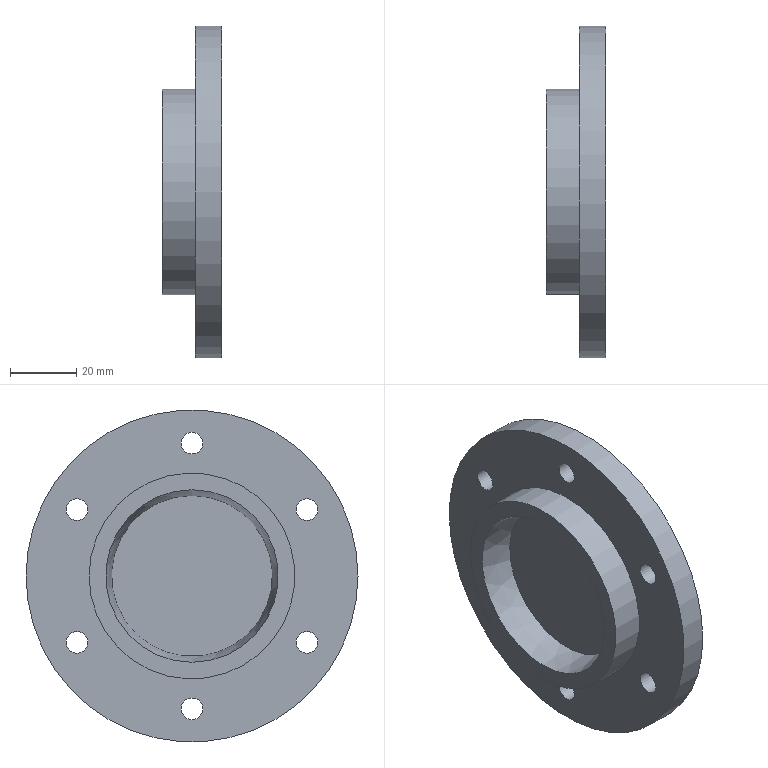Component | NX | DADUANMENGAI | 1 solid | 13 faces | box 18 x 100 x 100 mm | volume 71600 mm3 | cylinder 8 | plane 4 | cone 1 | commonest cylinder face diameters 6.5 x6 100 x1 62 x1
STEP:
#1=CARTESIAN_POINT('',(0.,0.,0.));
#2=DIRECTION('',(0.,0.,1.));
#3=DIRECTION('',(1.,0.,0.));
#4=AXIS2_PLACEMENT_3D('',#1,#2,#3);
#5=CARTESIAN_POINT('',(111.,234.641,-71.25));
#6=VERTEX_POINT('',#5);
#7=CARTESIAN_POINT('',(111.,234.641,-64.75));
#8=VERTEX_POINT('',#7);
#9=CARTESIAN_POINT('',(111.,234.641,-68.));
#10=DIRECTION('',(1.,0.,0.));
#11=DIRECTION('',(0.,0.,-1.));
#12=AXIS2_PLACEMENT_3D('',#9,#10,#11);
#13=CIRCLE('',#12,3.25);
#14=CARTESIAN_POINT('',(111.,200.,-88.));
#15=DIRECTION('',(1.,0.,0.));
#16=DIRECTION('',(0.,0.,-1.));
#17=AXIS2_PLACEMENT_3D('',#14,#15,#16);
#18=PLANE('',#17);
#19=CARTESIAN_POINT('',(-20.,34.641));
#20=DIRECTION('',(1.,0.));
#21=AXIS2_PLACEMENT_2D('',#19,#20);
#22=CIRCLE('',#21,3.25);
#23=(GEOMETRIC_REPRESENTATION_CONTEXT(2)PARAMETRIC_REPRESENTATION_CONTEXT()REPRESENTATION_CONTEXT('',''));
#24=DEFINITIONAL_REPRESENTATION('',(#22),#23);
#25=PCURVE('',#18,#24);
#26=CARTESIAN_POINT('',(119.,234.641,-68.));
#27=DIRECTION('',(-1.,0.,0.));
#28=DIRECTION('',(0.,0.,1.));
#29=AXIS2_PLACEMENT_3D('',#26,#27,#28);
#30=CYLINDRICAL_SURFACE('',#29,3.25);
#31=CARTESIAN_POINT('',(3.142,8.));
#32=DIRECTION('',(-1.,0.));
#33=VECTOR('',#32,1.);
#34=LINE('',#31,#33);
#35=(GEOMETRIC_REPRESENTATION_CONTEXT(2)PARAMETRIC_REPRESENTATION_CONTEXT()REPRESENTATION_CONTEXT('',''));
#36=DEFINITIONAL_REPRESENTATION('',(#34),#35);
#37=PCURVE('',#30,#36);
#38=SURFACE_CURVE('',#13,(#25,#37),.PCURVE_S1.);
#39=EDGE_CURVE('',#6,#8,#38,.T.);
#40=ORIENTED_EDGE('',*,*,#39,.T.);
#41=CARTESIAN_POINT('',(111.,234.641,-68.));
#42=DIRECTION('',(1.,0.,0.));
#43=DIRECTION('',(0.,0.,-1.));
#44=AXIS2_PLACEMENT_3D('',#41,#42,#43);
#45=CIRCLE('',#44,3.25);
#46=CARTESIAN_POINT('',(-20.,34.641));
#47=DIRECTION('',(1.,0.));
#48=AXIS2_PLACEMENT_2D('',#46,#47);
#49=CIRCLE('',#48,3.25);
#50=(GEOMETRIC_REPRESENTATION_CONTEXT(2)PARAMETRIC_REPRESENTATION_CONTEXT()REPRESENTATION_CONTEXT('',''));
#51=DEFINITIONAL_REPRESENTATION('',(#49),#50);
#52=PCURVE('',#18,#51);
#53=CARTESIAN_POINT('',(9.425,8.));
#54=DIRECTION('',(-1.,0.));
#55=VECTOR('',#54,1.);
#56=LINE('',#53,#55);
#57=(GEOMETRIC_REPRESENTATION_CONTEXT(2)PARAMETRIC_REPRESENTATION_CONTEXT()REPRESENTATION_CONTEXT('',''));
#58=DEFINITIONAL_REPRESENTATION('',(#56),#57);
#59=PCURVE('',#30,#58);
#60=SURFACE_CURVE('',#45,(#52,#59),.PCURVE_S1.);
#61=EDGE_CURVE('',#8,#6,#60,.T.);
#62=ORIENTED_EDGE('',*,*,#61,.T.);
#63=EDGE_LOOP('',(#40,#62));
#64=FACE_BOUND('',#63,.T.);
#65=CARTESIAN_POINT('',(111.,234.641,-111.25));
#66=VERTEX_POINT('',#65);
#67=CARTESIAN_POINT('',(111.,234.641,-104.75));
#68=VERTEX_POINT('',#67);
#69=CARTESIAN_POINT('',(111.,234.641,-108.));
#70=DIRECTION('',(1.,0.,0.));
#71=DIRECTION('',(0.,0.,-1.));
#72=AXIS2_PLACEMENT_3D('',#69,#70,#71);
#73=CIRCLE('',#72,3.25);
#74=CARTESIAN_POINT('',(20.,34.641));
#75=DIRECTION('',(1.,0.));
#76=AXIS2_PLACEMENT_2D('',#74,#75);
#77=CIRCLE('',#76,3.25);
#78=(GEOMETRIC_REPRESENTATION_CONTEXT(2)PARAMETRIC_REPRESENTATION_CONTEXT()REPRESENTATION_CONTEXT('',''));
#79=DEFINITIONAL_REPRESENTATION('',(#77),#78);
#80=PCURVE('',#18,#79);
#81=CARTESIAN_POINT('',(119.,234.641,-108.));
#82=DIRECTION('',(-1.,0.,0.));
#83=DIRECTION('',(0.,0.,1.));
#84=AXIS2_PLACEMENT_3D('',#81,#82,#83);
#85=CYLINDRICAL_SURFACE('',#84,3.25);
#86=CARTESIAN_POINT('',(3.142,8.));
#87=DIRECTION('',(-1.,0.));
#88=VECTOR('',#87,1.);
#89=LINE('',#86,#88);
#90=(GEOMETRIC_REPRESENTATION_CONTEXT(2)PARAMETRIC_REPRESENTATION_CONTEXT()REPRESENTATION_CONTEXT('',''));
#91=DEFINITIONAL_REPRESENTATION('',(#89),#90);
#92=PCURVE('',#85,#91);
#93=SURFACE_CURVE('',#73,(#80,#92),.PCURVE_S1.);
#94=EDGE_CURVE('',#66,#68,#93,.T.);
#95=ORIENTED_EDGE('',*,*,#94,.T.);
#96=CARTESIAN_POINT('',(111.,234.641,-108.));
#97=DIRECTION('',(1.,0.,0.));
#98=DIRECTION('',(0.,0.,-1.));
#99=AXIS2_PLACEMENT_3D('',#96,#97,#98);
#100=CIRCLE('',#99,3.25);
#101=CARTESIAN_POINT('',(20.,34.641));
#102=DIRECTION('',(1.,0.));
#103=AXIS2_PLACEMENT_2D('',#101,#102);
#104=CIRCLE('',#103,3.25);
#105=(GEOMETRIC_REPRESENTATION_CONTEXT(2)PARAMETRIC_REPRESENTATION_CONTEXT()REPRESENTATION_CONTEXT('',''));
#106=DEFINITIONAL_REPRESENTATION('',(#104),#105);
#107=PCURVE('',#18,#106);
#108=CARTESIAN_POINT('',(9.425,8.));
#109=DIRECTION('',(-1.,0.));
#110=VECTOR('',#109,1.);
#111=LINE('',#108,#110);
#112=(GEOMETRIC_REPRESENTATION_CONTEXT(2)PARAMETRIC_REPRESENTATION_CONTEXT()REPRESENTATION_CONTEXT('',''));
#113=DEFINITIONAL_REPRESENTATION('',(#111),#112);
#114=PCURVE('',#85,#113);
#115=SURFACE_CURVE('',#100,(#107,#114),.PCURVE_S1.);
#116=EDGE_CURVE('',#68,#66,#115,.T.);
#117=ORIENTED_EDGE('',*,*,#116,.T.);
#118=EDGE_LOOP('',(#95,#117));
#119=FACE_BOUND('',#118,.T.);
#120=CARTESIAN_POINT('',(111.,200.,-51.25));
#121=VERTEX_POINT('',#120);
#122=CARTESIAN_POINT('',(111.,200.,-44.75));
#123=VERTEX_POINT('',#122);
#124=CARTESIAN_POINT('',(111.,200.,-48.));
#125=DIRECTION('',(1.,0.,0.));
#126=DIRECTION('',(0.,0.,-1.));
#127=AXIS2_PLACEMENT_3D('',#124,#125,#126);
#128=CIRCLE('',#127,3.25);
#129=CARTESIAN_POINT('',(-40.,0.));
#130=DIRECTION('',(1.,0.));
#131=AXIS2_PLACEMENT_2D('',#129,#130);
#132=CIRCLE('',#131,3.25);
#133=(GEOMETRIC_REPRESENTATION_CONTEXT(2)PARAMETRIC_REPRESENTATION_CONTEXT()REPRESENTATION_CONTEXT('',''));
#134=DEFINITIONAL_REPRESENTATION('',(#132),#133);
#135=PCURVE('',#18,#134);
#136=CARTESIAN_POINT('',(119.,200.,-48.));
#137=DIRECTION('',(-1.,0.,0.));
#138=DIRECTION('',(0.,0.,1.));
#139=AXIS2_PLACEMENT_3D('',#136,#137,#138);
#140=CYLINDRICAL_SURFACE('',#139,3.25);
#141=CARTESIAN_POINT('',(3.142,8.));
#142=DIRECTION('',(-1.,0.));
#143=VECTOR('',#142,1.);
#144=LINE('',#141,#143);
#145=(GEOMETRIC_REPRESENTATION_CONTEXT(2)PARAMETRIC_REPRESENTATION_CONTEXT()REPRESENTATION_CONTEXT('',''));
#146=DEFINITIONAL_REPRESENTATION('',(#144),#145);
#147=PCURVE('',#140,#146);
#148=SURFACE_CURVE('',#128,(#135,#147),.PCURVE_S1.);
#149=EDGE_CURVE('',#121,#123,#148,.T.);
#150=ORIENTED_EDGE('',*,*,#149,.T.);
#151=CARTESIAN_POINT('',(111.,200.,-48.));
#152=DIRECTION('',(1.,0.,0.));
#153=DIRECTION('',(0.,0.,-1.));
#154=AXIS2_PLACEMENT_3D('',#151,#152,#153);
#155=CIRCLE('',#154,3.25);
#156=CARTESIAN_POINT('',(-40.,0.));
#157=DIRECTION('',(1.,0.));
#158=AXIS2_PLACEMENT_2D('',#156,#157);
#159=CIRCLE('',#158,3.25);
#160=(GEOMETRIC_REPRESENTATION_CONTEXT(2)PARAMETRIC_REPRESENTATION_CONTEXT()REPRESENTATION_CONTEXT('',''));
#161=DEFINITIONAL_REPRESENTATION('',(#159),#160);
#162=PCURVE('',#18,#161);
#163=CARTESIAN_POINT('',(9.425,8.));
#164=DIRECTION('',(-1.,0.));
#165=VECTOR('',#164,1.);
#166=LINE('',#163,#165);
#167=(GEOMETRIC_REPRESENTATION_CONTEXT(2)PARAMETRIC_REPRESENTATION_CONTEXT()REPRESENTATION_CONTEXT('',''));
#168=DEFINITIONAL_REPRESENTATION('',(#166),#167);
#169=PCURVE('',#140,#168);
#170=SURFACE_CURVE('',#155,(#162,#169),.PCURVE_S1.);
#171=EDGE_CURVE('',#123,#121,#170,.T.);
#172=ORIENTED_EDGE('',*,*,#171,.T.);
#173=EDGE_LOOP('',(#150,#172));
#174=FACE_BOUND('',#173,.T.);
#175=CARTESIAN_POINT('',(111.,200.,-131.25));
#176=VERTEX_POINT('',#175);
#177=CARTESIAN_POINT('',(111.,200.,-124.75));
#178=VERTEX_POINT('',#177);
#179=CARTESIAN_POINT('',(111.,200.,-128.));
#180=DIRECTION('',(1.,0.,0.));
#181=DIRECTION('',(0.,0.,-1.));
#182=AXIS2_PLACEMENT_3D('',#179,#180,#181);
#183=CIRCLE('',#182,3.25);
#184=CARTESIAN_POINT('',(40.,0.));
#185=DIRECTION('',(1.,0.));
#186=AXIS2_PLACEMENT_2D('',#184,#185);
#187=CIRCLE('',#186,3.25);
#188=(GEOMETRIC_REPRESENTATION_CONTEXT(2)PARAMETRIC_REPRESENTATION_CONTEXT()REPRESENTATION_CONTEXT('',''));
#189=DEFINITIONAL_REPRESENTATION('',(#187),#188);
#190=PCURVE('',#18,#189);
#191=CARTESIAN_POINT('',(119.,200.,-128.));
#192=DIRECTION('',(-1.,0.,0.));
#193=DIRECTION('',(0.,0.,1.));
#194=AXIS2_PLACEMENT_3D('',#191,#192,#193);
#195=CYLINDRICAL_SURFACE('',#194,3.25);
#196=CARTESIAN_POINT('',(3.142,8.));
#197=DIRECTION('',(-1.,0.));
#198=VECTOR('',#197,1.);
#199=LINE('',#196,#198);
#200=(GEOMETRIC_REPRESENTATION_CONTEXT(2)PARAMETRIC_REPRESENTATION_CONTEXT()REPRESENTATION_CONTEXT('',''));
#201=DEFINITIONAL_REPRESENTATION('',(#199),#200);
#202=PCURVE('',#195,#201);
#203=SURFACE_CURVE('',#183,(#190,#202),.PCURVE_S1.);
#204=EDGE_CURVE('',#176,#178,#203,.T.);
#205=ORIENTED_EDGE('',*,*,#204,.T.);
#206=CARTESIAN_POINT('',(111.,200.,-128.));
#207=DIRECTION('',(1.,0.,0.));
#208=DIRECTION('',(0.,0.,-1.));
#209=AXIS2_PLACEMENT_3D('',#206,#207,#208);
#210=CIRCLE('',#209,3.25);
#211=CARTESIAN_POINT('',(40.,0.));
#212=DIRECTION('',(1.,0.));
#213=AXIS2_PLACEMENT_2D('',#211,#212);
#214=CIRCLE('',#213,3.25);
#215=(GEOMETRIC_REPRESENTATION_CONTEXT(2)PARAMETRIC_REPRESENTATION_CONTEXT()REPRESENTATION_CONTEXT('',''));
#216=DEFINITIONAL_REPRESENTATION('',(#214),#215);
#217=PCURVE('',#18,#216);
#218=CARTESIAN_POINT('',(9.425,8.));
#219=DIRECTION('',(-1.,0.));
#220=VECTOR('',#219,1.);
#221=LINE('',#218,#220);
#222=(GEOMETRIC_REPRESENTATION_CONTEXT(2)PARAMETRIC_REPRESENTATION_CONTEXT()REPRESENTATION_CONTEXT('',''));
#223=DEFINITIONAL_REPRESENTATION('',(#221),#222);
#224=PCURVE('',#195,#223);
#225=SURFACE_CURVE('',#210,(#217,#224),.PCURVE_S1.);
#226=EDGE_CURVE('',#178,#176,#225,.T.);
#227=ORIENTED_EDGE('',*,*,#226,.T.);
#228=EDGE_LOOP('',(#205,#227));
#229=FACE_BOUND('',#228,.T.);
#230=CARTESIAN_POINT('',(111.,165.359,-71.25));
#231=VERTEX_POINT('',#230);
#232=CARTESIAN_POINT('',(111.,165.359,-64.75));
#233=VERTEX_POINT('',#232);
#234=CARTESIAN_POINT('',(111.,165.359,-68.));
#235=DIRECTION('',(1.,0.,0.));
#236=DIRECTION('',(0.,0.,-1.));
#237=AXIS2_PLACEMENT_3D('',#234,#235,#236);
#238=CIRCLE('',#237,3.25);
#239=CARTESIAN_POINT('',(-20.,-34.641));
#240=DIRECTION('',(1.,0.));
#241=AXIS2_PLACEMENT_2D('',#239,#240);
#242=CIRCLE('',#241,3.25);
#243=(GEOMETRIC_REPRESENTATION_CONTEXT(2)PARAMETRIC_REPRESENTATION_CONTEXT()REPRESENTATION_CONTEXT('',''));
#244=DEFINITIONAL_REPRESENTATION('',(#242),#243);
#245=PCURVE('',#18,#244);
#246=CARTESIAN_POINT('',(119.,165.359,-68.));
#247=DIRECTION('',(-1.,0.,0.));
#248=DIRECTION('',(0.,0.,1.));
#249=AXIS2_PLACEMENT_3D('',#246,#247,#248);
#250=CYLINDRICAL_SURFACE('',#249,3.25);
#251=CARTESIAN_POINT('',(3.142,8.));
#252=DIRECTION('',(-1.,0.));
#253=VECTOR('',#252,1.);
#254=LINE('',#251,#253);
#255=(GEOMETRIC_REPRESENTATION_CONTEXT(2)PARAMETRIC_REPRESENTATION_CONTEXT()REPRESENTATION_CONTEXT('',''));
#256=DEFINITIONAL_REPRESENTATION('',(#254),#255);
#257=PCURVE('',#250,#256);
#258=SURFACE_CURVE('',#238,(#245,#257),.PCURVE_S1.);
#259=EDGE_CURVE('',#231,#233,#258,.T.);
#260=ORIENTED_EDGE('',*,*,#259,.T.);
#261=CARTESIAN_POINT('',(111.,165.359,-68.));
#262=DIRECTION('',(1.,0.,0.));
#263=DIRECTION('',(0.,0.,-1.));
#264=AXIS2_PLACEMENT_3D('',#261,#262,#263);
#265=CIRCLE('',#264,3.25);
#266=CARTESIAN_POINT('',(-20.,-34.641));
#267=DIRECTION('',(1.,0.));
#268=AXIS2_PLACEMENT_2D('',#266,#267);
#269=CIRCLE('',#268,3.25);
#270=(GEOMETRIC_REPRESENTATION_CONTEXT(2)PARAMETRIC_REPRESENTATION_CONTEXT()REPRESENTATION_CONTEXT('',''));
#271=DEFINITIONAL_REPRESENTATION('',(#269),#270);
#272=PCURVE('',#18,#271);
#273=CARTESIAN_POINT('',(9.425,8.));
#274=DIRECTION('',(-1.,0.));
#275=VECTOR('',#274,1.);
#276=LINE('',#273,#275);
#277=(GEOMETRIC_REPRESENTATION_CONTEXT(2)PARAMETRIC_REPRESENTATION_CONTEXT()REPRESENTATION_CONTEXT('',''));
#278=DEFINITIONAL_REPRESENTATION('',(#276),#277);
#279=PCURVE('',#250,#278);
#280=SURFACE_CURVE('',#265,(#272,#279),.PCURVE_S1.);
#281=EDGE_CURVE('',#233,#231,#280,.T.);
#282=ORIENTED_EDGE('',*,*,#281,.T.);
#283=EDGE_LOOP('',(#260,#282));
#284=FACE_BOUND('',#283,.T.);
#285=CARTESIAN_POINT('',(111.,165.359,-111.25));
#286=VERTEX_POINT('',#285);
#287=CARTESIAN_POINT('',(111.,165.359,-104.75));
#288=VERTEX_POINT('',#287);
#289=CARTESIAN_POINT('',(111.,165.359,-108.));
#290=DIRECTION('',(1.,0.,0.));
#291=DIRECTION('',(0.,0.,-1.));
#292=AXIS2_PLACEMENT_3D('',#289,#290,#291);
#293=CIRCLE('',#292,3.25);
#294=CARTESIAN_POINT('',(20.,-34.641));
#295=DIRECTION('',(1.,0.));
#296=AXIS2_PLACEMENT_2D('',#294,#295);
#297=CIRCLE('',#296,3.25);
#298=(GEOMETRIC_REPRESENTATION_CONTEXT(2)PARAMETRIC_REPRESENTATION_CONTEXT()REPRESENTATION_CONTEXT('',''));
#299=DEFINITIONAL_REPRESENTATION('',(#297),#298);
#300=PCURVE('',#18,#299);
#301=CARTESIAN_POINT('',(119.,165.359,-108.));
#302=DIRECTION('',(-1.,0.,0.));
#303=DIRECTION('',(0.,0.,1.));
#304=AXIS2_PLACEMENT_3D('',#301,#302,#303);
#305=CYLINDRICAL_SURFACE('',#304,3.25);
#306=CARTESIAN_POINT('',(3.142,8.));
#307=DIRECTION('',(-1.,0.));
#308=VECTOR('',#307,1.);
#309=LINE('',#306,#308);
#310=(GEOMETRIC_REPRESENTATION_CONTEXT(2)PARAMETRIC_REPRESENTATION_CONTEXT()REPRESENTATION_CONTEXT('',''));
#311=DEFINITIONAL_REPRESENTATION('',(#309),#310);
#312=PCURVE('',#305,#311);
#313=SURFACE_CURVE('',#293,(#300,#312),.PCURVE_S1.);
#314=EDGE_CURVE('',#286,#288,#313,.T.);
#315=ORIENTED_EDGE('',*,*,#314,.T.);
#316=CARTESIAN_POINT('',(111.,165.359,-108.));
#317=DIRECTION('',(1.,0.,0.));
#318=DIRECTION('',(0.,0.,-1.));
#319=AXIS2_PLACEMENT_3D('',#316,#317,#318);
#320=CIRCLE('',#319,3.25);
#321=CARTESIAN_POINT('',(20.,-34.641));
#322=DIRECTION('',(1.,0.));
#323=AXIS2_PLACEMENT_2D('',#321,#322);
#324=CIRCLE('',#323,3.25);
#325=(GEOMETRIC_REPRESENTATION_CONTEXT(2)PARAMETRIC_REPRESENTATION_CONTEXT()REPRESENTATION_CONTEXT('',''));
#326=DEFINITIONAL_REPRESENTATION('',(#324),#325);
#327=PCURVE('',#18,#326);
#328=CARTESIAN_POINT('',(9.425,8.));
#329=DIRECTION('',(-1.,0.));
#330=VECTOR('',#329,1.);
#331=LINE('',#328,#330);
#332=(GEOMETRIC_REPRESENTATION_CONTEXT(2)PARAMETRIC_REPRESENTATION_CONTEXT()REPRESENTATION_CONTEXT('',''));
#333=DEFINITIONAL_REPRESENTATION('',(#331),#332);
#334=PCURVE('',#305,#333);
#335=SURFACE_CURVE('',#320,(#327,#334),.PCURVE_S1.);
#336=EDGE_CURVE('',#288,#286,#335,.T.);
#337=ORIENTED_EDGE('',*,*,#336,.T.);
#338=EDGE_LOOP('',(#315,#337));
#339=FACE_BOUND('',#338,.T.);
#340=CARTESIAN_POINT('',(111.,250.,-88.));
#341=VERTEX_POINT('',#340);
#342=CARTESIAN_POINT('',(111.,200.,-88.));
#343=DIRECTION('',(1.,0.,0.));
#344=DIRECTION('',(0.,1.,0.));
#345=AXIS2_PLACEMENT_3D('',#342,#343,#344);
#346=CIRCLE('',#345,50.);
#347=CARTESIAN_POINT('',(0.,0.));
#348=DIRECTION('',(0.,1.));
#349=AXIS2_PLACEMENT_2D('',#347,#348);
#350=CIRCLE('',#349,50.);
#351=(GEOMETRIC_REPRESENTATION_CONTEXT(2)PARAMETRIC_REPRESENTATION_CONTEXT()REPRESENTATION_CONTEXT('',''));
#352=DEFINITIONAL_REPRESENTATION('',(#350),#351);
#353=PCURVE('',#18,#352);
#354=CARTESIAN_POINT('',(119.,200.,-88.));
#355=DIRECTION('',(-1.,0.,0.));
#356=DIRECTION('',(0.,0.,1.));
#357=AXIS2_PLACEMENT_3D('',#354,#355,#356);
#358=CYLINDRICAL_SURFACE('',#357,50.);
#359=CARTESIAN_POINT('',(7.854,8.));
#360=DIRECTION('',(-1.,0.));
#361=VECTOR('',#360,1.);
#362=LINE('',#359,#361);
#363=(GEOMETRIC_REPRESENTATION_CONTEXT(2)PARAMETRIC_REPRESENTATION_CONTEXT()REPRESENTATION_CONTEXT('',''));
#364=DEFINITIONAL_REPRESENTATION('',(#362),#363);
#365=PCURVE('',#358,#364);
#366=SURFACE_CURVE('',#346,(#353,#365),.PCURVE_S1.);
#367=EDGE_CURVE('',#341,#341,#366,.T.);
#368=ORIENTED_EDGE('',*,*,#367,.F.);
#369=EDGE_LOOP('',(#368));
#370=FACE_BOUND('',#369,.T.);
#371=CARTESIAN_POINT('',(111.,231.,-88.));
#372=VERTEX_POINT('',#371);
#373=CARTESIAN_POINT('',(111.,200.,-88.));
#374=DIRECTION('',(-1.,0.,0.));
#375=DIRECTION('',(0.,1.,0.));
#376=AXIS2_PLACEMENT_3D('',#373,#374,#375);
#377=CIRCLE('',#376,31.);
#378=CARTESIAN_POINT('',(0.,31.));
#379=CARTESIAN_POINT('',(53.694,31.));
#380=CARTESIAN_POINT('',(26.847,-15.5));
#381=CARTESIAN_POINT('',(0.,-62.));
#382=CARTESIAN_POINT('',(-26.847,-15.5));
#383=CARTESIAN_POINT('',(-53.694,31.));
#384=CARTESIAN_POINT('',(0.,31.));
#385=(BOUNDED_CURVE()B_SPLINE_CURVE(2,(#378,#379,#380,#381,#382,#383,#384),.UNSPECIFIED.,.T.,.F.)B_SPLINE_CURVE_WITH_KNOTS((1,2,2,2,2,1),(-2.094,0.,2.094,4.189,6.283,8.378),.UNSPECIFIED.)CURVE()GEOMETRIC_REPRESENTATION_ITEM()RATIONAL_B_SPLINE_CURVE((1.,0.5,1.,0.5,1.,0.5,1.))REPRESENTATION_ITEM(''));
#386=(GEOMETRIC_REPRESENTATION_CONTEXT(2)PARAMETRIC_REPRESENTATION_CONTEXT()REPRESENTATION_CONTEXT('',''));
#387=DEFINITIONAL_REPRESENTATION('',(#385),#386);
#388=PCURVE('',#18,#387);
#389=CARTESIAN_POINT('',(101.,200.,-88.));
#390=DIRECTION('',(1.,0.,0.));
#391=DIRECTION('',(0.,0.,-1.));
#392=AXIS2_PLACEMENT_3D('',#389,#390,#391);
#393=CYLINDRICAL_SURFACE('',#392,31.);
#394=CARTESIAN_POINT('',(7.854,10.));
#395=DIRECTION('',(-1.,0.));
#396=VECTOR('',#395,1.);
#397=LINE('',#394,#396);
#398=(GEOMETRIC_REPRESENTATION_CONTEXT(2)PARAMETRIC_REPRESENTATION_CONTEXT()REPRESENTATION_CONTEXT('',''));
#399=DEFINITIONAL_REPRESENTATION('',(#397),#398);
#400=PCURVE('',#393,#399);
#401=SURFACE_CURVE('',#377,(#388,#400),.PCURVE_S1.);
#402=EDGE_CURVE('',#372,#372,#401,.T.);
#403=ORIENTED_EDGE('',*,*,#402,.F.);
#404=EDGE_LOOP('',(#403));
#405=FACE_BOUND('',#404,.T.);
#406=ADVANCED_FACE('',(#64,#119,#174,#229,#284,#339,#370,#405),#18,.F.);
#407=CARTESIAN_POINT('',(119.,250.,-88.));
#408=VERTEX_POINT('',#407);
#409=CARTESIAN_POINT('',(119.,200.,-88.));
#410=DIRECTION('',(1.,0.,0.));
#411=DIRECTION('',(0.,1.,0.));
#412=AXIS2_PLACEMENT_3D('',#409,#410,#411);
#413=CIRCLE('',#412,50.);
#414=CARTESIAN_POINT('',(7.854,0.));
#415=DIRECTION('',(-1.,0.));
#416=VECTOR('',#415,1.);
#417=LINE('',#414,#416);
#418=(GEOMETRIC_REPRESENTATION_CONTEXT(2)PARAMETRIC_REPRESENTATION_CONTEXT()REPRESENTATION_CONTEXT('',''));
#419=DEFINITIONAL_REPRESENTATION('',(#417),#418);
#420=PCURVE('',#358,#419);
#421=CARTESIAN_POINT('',(119.,200.,-88.));
#422=DIRECTION('',(1.,0.,0.));
#423=DIRECTION('',(0.,0.,-1.));
#424=AXIS2_PLACEMENT_3D('',#421,#422,#423);
#425=PLANE('',#424);
#426=CARTESIAN_POINT('',(0.,0.));
#427=DIRECTION('',(0.,1.));
#428=AXIS2_PLACEMENT_2D('',#426,#427);
#429=CIRCLE('',#428,50.);
#430=(GEOMETRIC_REPRESENTATION_CONTEXT(2)PARAMETRIC_REPRESENTATION_CONTEXT()REPRESENTATION_CONTEXT('',''));
#431=DEFINITIONAL_REPRESENTATION('',(#429),#430);
#432=PCURVE('',#425,#431);
#433=SURFACE_CURVE('',#413,(#420,#432),.PCURVE_S1.);
#434=EDGE_CURVE('',#408,#408,#433,.T.);
#435=ORIENTED_EDGE('',*,*,#434,.F.);
#436=CARTESIAN_POINT('',(119.,250.,-88.));
#437=CARTESIAN_POINT('',(111.,250.,-88.));
#438=B_SPLINE_CURVE_WITH_KNOTS('',1,(#436,#437),.UNSPECIFIED.,.F.,.F.,(2,2),(0.,8.),.PIECEWISE_BEZIER_KNOTS.);
#439=CARTESIAN_POINT('',(7.854,0.));
#440=DIRECTION('',(0.,1.));
#441=VECTOR('',#440,1.);
#442=LINE('',#439,#441);
#443=(GEOMETRIC_REPRESENTATION_CONTEXT(2)PARAMETRIC_REPRESENTATION_CONTEXT()REPRESENTATION_CONTEXT('',''));
#444=DEFINITIONAL_REPRESENTATION('',(#442),#443);
#445=PCURVE('',#358,#444);
#446=CARTESIAN_POINT('',(1.571,0.));
#447=DIRECTION('',(0.,1.));
#448=VECTOR('',#447,1.);
#449=LINE('',#446,#448);
#450=(GEOMETRIC_REPRESENTATION_CONTEXT(2)PARAMETRIC_REPRESENTATION_CONTEXT()REPRESENTATION_CONTEXT('',''));
#451=DEFINITIONAL_REPRESENTATION('',(#449),#450);
#452=PCURVE('',#358,#451);
#453=SEAM_CURVE('',#438,(#445,#452),.PCURVE_S1.);
#454=EDGE_CURVE('',#408,#341,#453,.T.);
#455=ORIENTED_EDGE('',*,*,#454,.T.);
#456=ORIENTED_EDGE('',*,*,#367,.T.);
#457=ORIENTED_EDGE('',*,*,#454,.F.);
#458=EDGE_LOOP('',(#435,#455,#456,#457));
#459=FACE_BOUND('',#458,.T.);
#460=ADVANCED_FACE('',(#459),#358,.T.);
#461=CARTESIAN_POINT('',(119.,234.641,-64.75));
#462=VERTEX_POINT('',#461);
#463=CARTESIAN_POINT('',(119.,234.641,-68.));
#464=DIRECTION('',(-1.,0.,0.));
#465=DIRECTION('',(0.,0.,1.));
#466=AXIS2_PLACEMENT_3D('',#463,#464,#465);
#467=CIRCLE('',#466,3.25);
#468=CARTESIAN_POINT('',(-23.25,34.641));
#469=CARTESIAN_POINT('',(-23.25,40.27));
#470=CARTESIAN_POINT('',(-18.375,37.456));
#471=CARTESIAN_POINT('',(-13.5,34.641));
#472=CARTESIAN_POINT('',(-18.375,31.826));
#473=CARTESIAN_POINT('',(-23.25,29.012));
#474=CARTESIAN_POINT('',(-23.25,34.641));
#475=(BOUNDED_CURVE()B_SPLINE_CURVE(2,(#468,#469,#470,#471,#472,#473,#474),.UNSPECIFIED.,.T.,.F.)B_SPLINE_CURVE_WITH_KNOTS((1,2,2,2,2,1),(-2.094,0.,2.094,4.189,6.283,8.378),.UNSPECIFIED.)CURVE()GEOMETRIC_REPRESENTATION_ITEM()RATIONAL_B_SPLINE_CURVE((1.,0.5,1.,0.5,1.,0.5,1.))REPRESENTATION_ITEM(''));
#476=(GEOMETRIC_REPRESENTATION_CONTEXT(2)PARAMETRIC_REPRESENTATION_CONTEXT()REPRESENTATION_CONTEXT('',''));
#477=DEFINITIONAL_REPRESENTATION('',(#475),#476);
#478=PCURVE('',#425,#477);
#479=CARTESIAN_POINT('',(0.,0.));
#480=DIRECTION('',(1.,0.));
#481=VECTOR('',#480,1.);
#482=LINE('',#479,#481);
#483=(GEOMETRIC_REPRESENTATION_CONTEXT(2)PARAMETRIC_REPRESENTATION_CONTEXT()REPRESENTATION_CONTEXT('',''));
#484=DEFINITIONAL_REPRESENTATION('',(#482),#483);
#485=PCURVE('',#30,#484);
#486=SURFACE_CURVE('',#467,(#478,#485),.PCURVE_S1.);
#487=EDGE_CURVE('',#462,#462,#486,.T.);
#488=ORIENTED_EDGE('',*,*,#487,.T.);
#489=EDGE_LOOP('',(#488));
#490=FACE_BOUND('',#489,.T.);
#491=CARTESIAN_POINT('',(119.,234.641,-104.75));
#492=VERTEX_POINT('',#491);
#493=CARTESIAN_POINT('',(119.,234.641,-108.));
#494=DIRECTION('',(-1.,0.,0.));
#495=DIRECTION('',(0.,0.,1.));
#496=AXIS2_PLACEMENT_3D('',#493,#494,#495);
#497=CIRCLE('',#496,3.25);
#498=CARTESIAN_POINT('',(16.75,34.641));
#499=CARTESIAN_POINT('',(16.75,40.27));
#500=CARTESIAN_POINT('',(21.625,37.456));
#501=CARTESIAN_POINT('',(26.5,34.641));
#502=CARTESIAN_POINT('',(21.625,31.826));
#503=CARTESIAN_POINT('',(16.75,29.012));
#504=CARTESIAN_POINT('',(16.75,34.641));
#505=(BOUNDED_CURVE()B_SPLINE_CURVE(2,(#498,#499,#500,#501,#502,#503,#504),.UNSPECIFIED.,.T.,.F.)B_SPLINE_CURVE_WITH_KNOTS((1,2,2,2,2,1),(-2.094,0.,2.094,4.189,6.283,8.378),.UNSPECIFIED.)CURVE()GEOMETRIC_REPRESENTATION_ITEM()RATIONAL_B_SPLINE_CURVE((1.,0.5,1.,0.5,1.,0.5,1.))REPRESENTATION_ITEM(''));
#506=(GEOMETRIC_REPRESENTATION_CONTEXT(2)PARAMETRIC_REPRESENTATION_CONTEXT()REPRESENTATION_CONTEXT('',''));
#507=DEFINITIONAL_REPRESENTATION('',(#505),#506);
#508=PCURVE('',#425,#507);
#509=CARTESIAN_POINT('',(0.,0.));
#510=DIRECTION('',(1.,0.));
#511=VECTOR('',#510,1.);
#512=LINE('',#509,#511);
#513=(GEOMETRIC_REPRESENTATION_CONTEXT(2)PARAMETRIC_REPRESENTATION_CONTEXT()REPRESENTATION_CONTEXT('',''));
#514=DEFINITIONAL_REPRESENTATION('',(#512),#513);
#515=PCURVE('',#85,#514);
#516=SURFACE_CURVE('',#497,(#508,#515),.PCURVE_S1.);
#517=EDGE_CURVE('',#492,#492,#516,.T.);
#518=ORIENTED_EDGE('',*,*,#517,.T.);
#519=EDGE_LOOP('',(#518));
#520=FACE_BOUND('',#519,.T.);
#521=CARTESIAN_POINT('',(119.,200.,-44.75));
#522=VERTEX_POINT('',#521);
#523=CARTESIAN_POINT('',(119.,200.,-48.));
#524=DIRECTION('',(-1.,0.,0.));
#525=DIRECTION('',(0.,0.,1.));
#526=AXIS2_PLACEMENT_3D('',#523,#524,#525);
#527=CIRCLE('',#526,3.25);
#528=CARTESIAN_POINT('',(-43.25,0.));
#529=CARTESIAN_POINT('',(-43.25,5.629));
#530=CARTESIAN_POINT('',(-38.375,2.815));
#531=CARTESIAN_POINT('',(-33.5,0.));
#532=CARTESIAN_POINT('',(-38.375,-2.815));
#533=CARTESIAN_POINT('',(-43.25,-5.629));
#534=CARTESIAN_POINT('',(-43.25,0.));
#535=(BOUNDED_CURVE()B_SPLINE_CURVE(2,(#528,#529,#530,#531,#532,#533,#534),.UNSPECIFIED.,.T.,.F.)B_SPLINE_CURVE_WITH_KNOTS((1,2,2,2,2,1),(-2.094,0.,2.094,4.189,6.283,8.378),.UNSPECIFIED.)CURVE()GEOMETRIC_REPRESENTATION_ITEM()RATIONAL_B_SPLINE_CURVE((1.,0.5,1.,0.5,1.,0.5,1.))REPRESENTATION_ITEM(''));
#536=(GEOMETRIC_REPRESENTATION_CONTEXT(2)PARAMETRIC_REPRESENTATION_CONTEXT()REPRESENTATION_CONTEXT('',''));
#537=DEFINITIONAL_REPRESENTATION('',(#535),#536);
#538=PCURVE('',#425,#537);
#539=CARTESIAN_POINT('',(0.,0.));
#540=DIRECTION('',(1.,0.));
#541=VECTOR('',#540,1.);
#542=LINE('',#539,#541);
#543=(GEOMETRIC_REPRESENTATION_CONTEXT(2)PARAMETRIC_REPRESENTATION_CONTEXT()REPRESENTATION_CONTEXT('',''));
#544=DEFINITIONAL_REPRESENTATION('',(#542),#543);
#545=PCURVE('',#140,#544);
#546=SURFACE_CURVE('',#527,(#538,#545),.PCURVE_S1.);
#547=EDGE_CURVE('',#522,#522,#546,.T.);
#548=ORIENTED_EDGE('',*,*,#547,.T.);
#549=EDGE_LOOP('',(#548));
#550=FACE_BOUND('',#549,.T.);
#551=CARTESIAN_POINT('',(119.,200.,-124.75));
#552=VERTEX_POINT('',#551);
#553=CARTESIAN_POINT('',(119.,200.,-128.));
#554=DIRECTION('',(-1.,0.,0.));
#555=DIRECTION('',(0.,0.,1.));
#556=AXIS2_PLACEMENT_3D('',#553,#554,#555);
#557=CIRCLE('',#556,3.25);
#558=CARTESIAN_POINT('',(36.75,0.));
#559=CARTESIAN_POINT('',(36.75,5.629));
#560=CARTESIAN_POINT('',(41.625,2.815));
#561=CARTESIAN_POINT('',(46.5,0.));
#562=CARTESIAN_POINT('',(41.625,-2.815));
#563=CARTESIAN_POINT('',(36.75,-5.629));
#564=CARTESIAN_POINT('',(36.75,0.));
#565=(BOUNDED_CURVE()B_SPLINE_CURVE(2,(#558,#559,#560,#561,#562,#563,#564),.UNSPECIFIED.,.T.,.F.)B_SPLINE_CURVE_WITH_KNOTS((1,2,2,2,2,1),(-2.094,0.,2.094,4.189,6.283,8.378),.UNSPECIFIED.)CURVE()GEOMETRIC_REPRESENTATION_ITEM()RATIONAL_B_SPLINE_CURVE((1.,0.5,1.,0.5,1.,0.5,1.))REPRESENTATION_ITEM(''));
#566=(GEOMETRIC_REPRESENTATION_CONTEXT(2)PARAMETRIC_REPRESENTATION_CONTEXT()REPRESENTATION_CONTEXT('',''));
#567=DEFINITIONAL_REPRESENTATION('',(#565),#566);
#568=PCURVE('',#425,#567);
#569=CARTESIAN_POINT('',(0.,0.));
#570=DIRECTION('',(1.,0.));
#571=VECTOR('',#570,1.);
#572=LINE('',#569,#571);
#573=(GEOMETRIC_REPRESENTATION_CONTEXT(2)PARAMETRIC_REPRESENTATION_CONTEXT()REPRESENTATION_CONTEXT('',''));
#574=DEFINITIONAL_REPRESENTATION('',(#572),#573);
#575=PCURVE('',#195,#574);
#576=SURFACE_CURVE('',#557,(#568,#575),.PCURVE_S1.);
#577=EDGE_CURVE('',#552,#552,#576,.T.);
#578=ORIENTED_EDGE('',*,*,#577,.T.);
#579=EDGE_LOOP('',(#578));
#580=FACE_BOUND('',#579,.T.);
#581=CARTESIAN_POINT('',(119.,165.359,-64.75));
#582=VERTEX_POINT('',#581);
#583=CARTESIAN_POINT('',(119.,165.359,-68.));
#584=DIRECTION('',(-1.,0.,0.));
#585=DIRECTION('',(0.,0.,1.));
#586=AXIS2_PLACEMENT_3D('',#583,#584,#585);
#587=CIRCLE('',#586,3.25);
#588=CARTESIAN_POINT('',(-23.25,-34.641));
#589=CARTESIAN_POINT('',(-23.25,-29.012));
#590=CARTESIAN_POINT('',(-18.375,-31.826));
#591=CARTESIAN_POINT('',(-13.5,-34.641));
#592=CARTESIAN_POINT('',(-18.375,-37.456));
#593=CARTESIAN_POINT('',(-23.25,-40.27));
#594=CARTESIAN_POINT('',(-23.25,-34.641));
#595=(BOUNDED_CURVE()B_SPLINE_CURVE(2,(#588,#589,#590,#591,#592,#593,#594),.UNSPECIFIED.,.T.,.F.)B_SPLINE_CURVE_WITH_KNOTS((1,2,2,2,2,1),(-2.094,0.,2.094,4.189,6.283,8.378),.UNSPECIFIED.)CURVE()GEOMETRIC_REPRESENTATION_ITEM()RATIONAL_B_SPLINE_CURVE((1.,0.5,1.,0.5,1.,0.5,1.))REPRESENTATION_ITEM(''));
#596=(GEOMETRIC_REPRESENTATION_CONTEXT(2)PARAMETRIC_REPRESENTATION_CONTEXT()REPRESENTATION_CONTEXT('',''));
#597=DEFINITIONAL_REPRESENTATION('',(#595),#596);
#598=PCURVE('',#425,#597);
#599=CARTESIAN_POINT('',(0.,0.));
#600=DIRECTION('',(1.,0.));
#601=VECTOR('',#600,1.);
#602=LINE('',#599,#601);
#603=(GEOMETRIC_REPRESENTATION_CONTEXT(2)PARAMETRIC_REPRESENTATION_CONTEXT()REPRESENTATION_CONTEXT('',''));
#604=DEFINITIONAL_REPRESENTATION('',(#602),#603);
#605=PCURVE('',#250,#604);
#606=SURFACE_CURVE('',#587,(#598,#605),.PCURVE_S1.);
#607=EDGE_CURVE('',#582,#582,#606,.T.);
#608=ORIENTED_EDGE('',*,*,#607,.T.);
#609=EDGE_LOOP('',(#608));
#610=FACE_BOUND('',#609,.T.);
#611=CARTESIAN_POINT('',(119.,165.359,-104.75));
#612=VERTEX_POINT('',#611);
#613=CARTESIAN_POINT('',(119.,165.359,-108.));
#614=DIRECTION('',(-1.,0.,0.));
#615=DIRECTION('',(0.,0.,1.));
#616=AXIS2_PLACEMENT_3D('',#613,#614,#615);
#617=CIRCLE('',#616,3.25);
#618=CARTESIAN_POINT('',(16.75,-34.641));
#619=CARTESIAN_POINT('',(16.75,-29.012));
#620=CARTESIAN_POINT('',(21.625,-31.826));
#621=CARTESIAN_POINT('',(26.5,-34.641));
#622=CARTESIAN_POINT('',(21.625,-37.456));
#623=CARTESIAN_POINT('',(16.75,-40.27));
#624=CARTESIAN_POINT('',(16.75,-34.641));
#625=(BOUNDED_CURVE()B_SPLINE_CURVE(2,(#618,#619,#620,#621,#622,#623,#624),.UNSPECIFIED.,.T.,.F.)B_SPLINE_CURVE_WITH_KNOTS((1,2,2,2,2,1),(-2.094,0.,2.094,4.189,6.283,8.378),.UNSPECIFIED.)CURVE()GEOMETRIC_REPRESENTATION_ITEM()RATIONAL_B_SPLINE_CURVE((1.,0.5,1.,0.5,1.,0.5,1.))REPRESENTATION_ITEM(''));
#626=(GEOMETRIC_REPRESENTATION_CONTEXT(2)PARAMETRIC_REPRESENTATION_CONTEXT()REPRESENTATION_CONTEXT('',''));
#627=DEFINITIONAL_REPRESENTATION('',(#625),#626);
#628=PCURVE('',#425,#627);
#629=CARTESIAN_POINT('',(0.,0.));
#630=DIRECTION('',(1.,0.));
#631=VECTOR('',#630,1.);
#632=LINE('',#629,#631);
#633=(GEOMETRIC_REPRESENTATION_CONTEXT(2)PARAMETRIC_REPRESENTATION_CONTEXT()REPRESENTATION_CONTEXT('',''));
#634=DEFINITIONAL_REPRESENTATION('',(#632),#633);
#635=PCURVE('',#305,#634);
#636=SURFACE_CURVE('',#617,(#628,#635),.PCURVE_S1.);
#637=EDGE_CURVE('',#612,#612,#636,.T.);
#638=ORIENTED_EDGE('',*,*,#637,.T.);
#639=EDGE_LOOP('',(#638));
#640=FACE_BOUND('',#639,.T.);
#641=ORIENTED_EDGE('',*,*,#434,.T.);
#642=EDGE_LOOP('',(#641));
#643=FACE_BOUND('',#642,.T.);
#644=ADVANCED_FACE('',(#490,#520,#550,#580,#610,#640,#643),#425,.T.);
#645=CARTESIAN_POINT('',(101.,231.,-88.));
#646=VERTEX_POINT('',#645);
#647=CARTESIAN_POINT('',(101.,200.,-88.));
#648=DIRECTION('',(-1.,0.,0.));
#649=DIRECTION('',(0.,1.,0.));
#650=AXIS2_PLACEMENT_3D('',#647,#648,#649);
#651=CIRCLE('',#650,31.);
#652=CARTESIAN_POINT('',(7.854,0.));
#653=DIRECTION('',(-1.,0.));
#654=VECTOR('',#653,1.);
#655=LINE('',#652,#654);
#656=(GEOMETRIC_REPRESENTATION_CONTEXT(2)PARAMETRIC_REPRESENTATION_CONTEXT()REPRESENTATION_CONTEXT('',''));
#657=DEFINITIONAL_REPRESENTATION('',(#655),#656);
#658=PCURVE('',#393,#657);
#659=CARTESIAN_POINT('',(101.,200.,-88.));
#660=DIRECTION('',(-1.,0.,0.));
#661=DIRECTION('',(0.,0.,1.));
#662=AXIS2_PLACEMENT_3D('',#659,#660,#661);
#663=PLANE('',#662);
#664=CARTESIAN_POINT('',(0.,0.));
#665=DIRECTION('',(0.,1.));
#666=AXIS2_PLACEMENT_2D('',#664,#665);
#667=CIRCLE('',#666,31.);
#668=(GEOMETRIC_REPRESENTATION_CONTEXT(2)PARAMETRIC_REPRESENTATION_CONTEXT()REPRESENTATION_CONTEXT('',''));
#669=DEFINITIONAL_REPRESENTATION('',(#667),#668);
#670=PCURVE('',#663,#669);
#671=SURFACE_CURVE('',#651,(#658,#670),.PCURVE_S1.);
#672=EDGE_CURVE('',#646,#646,#671,.T.);
#673=ORIENTED_EDGE('',*,*,#672,.F.);
#674=CARTESIAN_POINT('',(101.,231.,-88.));
#675=CARTESIAN_POINT('',(111.,231.,-88.));
#676=B_SPLINE_CURVE_WITH_KNOTS('',1,(#674,#675),.UNSPECIFIED.,.F.,.F.,(2,2),(0.,10.),.PIECEWISE_BEZIER_KNOTS.);
#677=CARTESIAN_POINT('',(7.854,0.));
#678=DIRECTION('',(0.,1.));
#679=VECTOR('',#678,1.);
#680=LINE('',#677,#679);
#681=(GEOMETRIC_REPRESENTATION_CONTEXT(2)PARAMETRIC_REPRESENTATION_CONTEXT()REPRESENTATION_CONTEXT('',''));
#682=DEFINITIONAL_REPRESENTATION('',(#680),#681);
#683=PCURVE('',#393,#682);
#684=CARTESIAN_POINT('',(1.571,0.));
#685=DIRECTION('',(0.,1.));
#686=VECTOR('',#685,1.);
#687=LINE('',#684,#686);
#688=(GEOMETRIC_REPRESENTATION_CONTEXT(2)PARAMETRIC_REPRESENTATION_CONTEXT()REPRESENTATION_CONTEXT('',''));
#689=DEFINITIONAL_REPRESENTATION('',(#687),#688);
#690=PCURVE('',#393,#689);
#691=SEAM_CURVE('',#676,(#683,#690),.PCURVE_S1.);
#692=EDGE_CURVE('',#646,#372,#691,.T.);
#693=ORIENTED_EDGE('',*,*,#692,.T.);
#694=ORIENTED_EDGE('',*,*,#402,.T.);
#695=ORIENTED_EDGE('',*,*,#692,.F.);
#696=EDGE_LOOP('',(#673,#693,#694,#695));
#697=FACE_BOUND('',#696,.T.);
#698=ADVANCED_FACE('',(#697),#393,.T.);
#699=CARTESIAN_POINT('',(101.,200.,-62.));
#700=VERTEX_POINT('',#699);
#701=CARTESIAN_POINT('',(101.,200.,-88.));
#702=DIRECTION('',(-1.,0.,0.));
#703=DIRECTION('',(0.,0.,1.));
#704=AXIS2_PLACEMENT_3D('',#701,#702,#703);
#705=CIRCLE('',#704,26.);
#706=CARTESIAN_POINT('',(0.,0.));
#707=DIRECTION('',(1.,0.));
#708=AXIS2_PLACEMENT_2D('',#706,#707);
#709=CIRCLE('',#708,26.);
#710=(GEOMETRIC_REPRESENTATION_CONTEXT(2)PARAMETRIC_REPRESENTATION_CONTEXT()REPRESENTATION_CONTEXT('',''));
#711=DEFINITIONAL_REPRESENTATION('',(#709),#710);
#712=PCURVE('',#663,#711);
#713=CARTESIAN_POINT('',(101.,200.,-88.));
#714=DIRECTION('',(-1.,0.,0.));
#715=DIRECTION('',(0.,0.,1.));
#716=AXIS2_PLACEMENT_3D('',#713,#714,#715);
#717=CONICAL_SURFACE('',#716,26.,0.1745);
#718=CARTESIAN_POINT('',(0.,0.));
#719=DIRECTION('',(1.,0.));
#720=VECTOR('',#719,1.);
#721=LINE('',#718,#720);
#722=(GEOMETRIC_REPRESENTATION_CONTEXT(2)PARAMETRIC_REPRESENTATION_CONTEXT()REPRESENTATION_CONTEXT('',''));
#723=DEFINITIONAL_REPRESENTATION('',(#721),#722);
#724=PCURVE('',#717,#723);
#725=SURFACE_CURVE('',#705,(#712,#724),.PCURVE_S1.);
#726=EDGE_CURVE('',#700,#700,#725,.T.);
#727=ORIENTED_EDGE('',*,*,#726,.F.);
#728=EDGE_LOOP('',(#727));
#729=FACE_BOUND('',#728,.T.);
#730=ORIENTED_EDGE('',*,*,#672,.T.);
#731=EDGE_LOOP('',(#730));
#732=FACE_BOUND('',#731,.T.);
#733=ADVANCED_FACE('',(#729,#732),#663,.T.);
#734=CARTESIAN_POINT('',(111.,200.,-63.763));
#735=VERTEX_POINT('',#734);
#736=CARTESIAN_POINT('',(111.,200.,-88.));
#737=DIRECTION('',(1.,0.,0.));
#738=DIRECTION('',(0.,0.,1.));
#739=AXIS2_PLACEMENT_3D('',#736,#737,#738);
#740=CIRCLE('',#739,24.237);
#741=CARTESIAN_POINT('',(6.283,-10.));
#742=DIRECTION('',(-1.,0.));
#743=VECTOR('',#742,1.);
#744=LINE('',#741,#743);
#745=(GEOMETRIC_REPRESENTATION_CONTEXT(2)PARAMETRIC_REPRESENTATION_CONTEXT()REPRESENTATION_CONTEXT('',''));
#746=DEFINITIONAL_REPRESENTATION('',(#744),#745);
#747=PCURVE('',#717,#746);
#748=CARTESIAN_POINT('',(111.,200.,-88.));
#749=DIRECTION('',(-1.,0.,0.));
#750=DIRECTION('',(0.,0.,1.));
#751=AXIS2_PLACEMENT_3D('',#748,#749,#750);
#752=PLANE('',#751);
#753=CARTESIAN_POINT('',(24.237,0.));
#754=CARTESIAN_POINT('',(24.237,-41.979));
#755=CARTESIAN_POINT('',(-12.118,-20.99));
#756=CARTESIAN_POINT('',(-48.473,-0.));
#757=CARTESIAN_POINT('',(-12.118,20.99));
#758=CARTESIAN_POINT('',(24.237,41.979));
#759=CARTESIAN_POINT('',(24.237,0.));
#760=(BOUNDED_CURVE()B_SPLINE_CURVE(2,(#753,#754,#755,#756,#757,#758,#759),.UNSPECIFIED.,.T.,.F.)B_SPLINE_CURVE_WITH_KNOTS((1,2,2,2,2,1),(-2.094,0.,2.094,4.189,6.283,8.378),.UNSPECIFIED.)CURVE()GEOMETRIC_REPRESENTATION_ITEM()RATIONAL_B_SPLINE_CURVE((1.,0.5,1.,0.5,1.,0.5,1.))REPRESENTATION_ITEM(''));
#761=(GEOMETRIC_REPRESENTATION_CONTEXT(2)PARAMETRIC_REPRESENTATION_CONTEXT()REPRESENTATION_CONTEXT('',''));
#762=DEFINITIONAL_REPRESENTATION('',(#760),#761);
#763=PCURVE('',#752,#762);
#764=SURFACE_CURVE('',#740,(#747,#763),.PCURVE_S1.);
#765=EDGE_CURVE('',#735,#735,#764,.T.);
#766=ORIENTED_EDGE('',*,*,#765,.F.);
#767=CARTESIAN_POINT('',(111.,200.,-63.763));
#768=CARTESIAN_POINT('',(101.,200.,-62.));
#769=B_SPLINE_CURVE_WITH_KNOTS('',1,(#767,#768),.UNSPECIFIED.,.F.,.F.,(2,2),(-10.154,0.),.PIECEWISE_BEZIER_KNOTS.);
#770=CARTESIAN_POINT('',(6.283,0.));
#771=DIRECTION('',(0.,1.));
#772=VECTOR('',#771,1.);
#773=LINE('',#770,#772);
#774=(GEOMETRIC_REPRESENTATION_CONTEXT(2)PARAMETRIC_REPRESENTATION_CONTEXT()REPRESENTATION_CONTEXT('',''));
#775=DEFINITIONAL_REPRESENTATION('',(#773),#774);
#776=PCURVE('',#717,#775);
#777=CARTESIAN_POINT('',(0.,0.));
#778=DIRECTION('',(0.,1.));
#779=VECTOR('',#778,1.);
#780=LINE('',#777,#779);
#781=(GEOMETRIC_REPRESENTATION_CONTEXT(2)PARAMETRIC_REPRESENTATION_CONTEXT()REPRESENTATION_CONTEXT('',''));
#782=DEFINITIONAL_REPRESENTATION('',(#780),#781);
#783=PCURVE('',#717,#782);
#784=SEAM_CURVE('',#769,(#776,#783),.PCURVE_S1.);
#785=EDGE_CURVE('',#735,#700,#784,.T.);
#786=ORIENTED_EDGE('',*,*,#785,.T.);
#787=ORIENTED_EDGE('',*,*,#726,.F.);
#788=ORIENTED_EDGE('',*,*,#785,.F.);
#789=EDGE_LOOP('',(#766,#786,#787,#788));
#790=FACE_BOUND('',#789,.F.);
#791=ADVANCED_FACE('',(#790),#717,.F.);
#792=ORIENTED_EDGE('',*,*,#765,.F.);
#793=EDGE_LOOP('',(#792));
#794=FACE_BOUND('',#793,.T.);
#795=ADVANCED_FACE('',(#794),#752,.T.);
#796=ORIENTED_EDGE('',*,*,#637,.T.);
#797=CARTESIAN_POINT('',(119.,165.359,-104.75));
#798=CARTESIAN_POINT('',(111.,165.359,-104.75));
#799=B_SPLINE_CURVE_WITH_KNOTS('',1,(#797,#798),.UNSPECIFIED.,.F.,.F.,(2,2),(0.,8.),.PIECEWISE_BEZIER_KNOTS.);
#800=CARTESIAN_POINT('',(6.283,0.));
#801=DIRECTION('',(0.,1.));
#802=VECTOR('',#801,1.);
#803=LINE('',#800,#802);
#804=(GEOMETRIC_REPRESENTATION_CONTEXT(2)PARAMETRIC_REPRESENTATION_CONTEXT()REPRESENTATION_CONTEXT('',''));
#805=DEFINITIONAL_REPRESENTATION('',(#803),#804);
#806=PCURVE('',#305,#805);
#807=CARTESIAN_POINT('',(0.,0.));
#808=DIRECTION('',(0.,1.));
#809=VECTOR('',#808,1.);
#810=LINE('',#807,#809);
#811=(GEOMETRIC_REPRESENTATION_CONTEXT(2)PARAMETRIC_REPRESENTATION_CONTEXT()REPRESENTATION_CONTEXT('',''));
#812=DEFINITIONAL_REPRESENTATION('',(#810),#811);
#813=PCURVE('',#305,#812);
#814=SEAM_CURVE('',#799,(#806,#813),.PCURVE_S1.);
#815=EDGE_CURVE('',#612,#288,#814,.T.);
#816=ORIENTED_EDGE('',*,*,#815,.T.);
#817=ORIENTED_EDGE('',*,*,#336,.T.);
#818=ORIENTED_EDGE('',*,*,#314,.T.);
#819=ORIENTED_EDGE('',*,*,#815,.F.);
#820=EDGE_LOOP('',(#796,#816,#817,#818,#819));
#821=FACE_BOUND('',#820,.F.);
#822=ADVANCED_FACE('',(#821),#305,.F.);
#823=ORIENTED_EDGE('',*,*,#607,.T.);
#824=CARTESIAN_POINT('',(119.,165.359,-64.75));
#825=CARTESIAN_POINT('',(111.,165.359,-64.75));
#826=B_SPLINE_CURVE_WITH_KNOTS('',1,(#824,#825),.UNSPECIFIED.,.F.,.F.,(2,2),(0.,8.),.PIECEWISE_BEZIER_KNOTS.);
#827=CARTESIAN_POINT('',(6.283,0.));
#828=DIRECTION('',(0.,1.));
#829=VECTOR('',#828,1.);
#830=LINE('',#827,#829);
#831=(GEOMETRIC_REPRESENTATION_CONTEXT(2)PARAMETRIC_REPRESENTATION_CONTEXT()REPRESENTATION_CONTEXT('',''));
#832=DEFINITIONAL_REPRESENTATION('',(#830),#831);
#833=PCURVE('',#250,#832);
#834=CARTESIAN_POINT('',(0.,0.));
#835=DIRECTION('',(0.,1.));
#836=VECTOR('',#835,1.);
#837=LINE('',#834,#836);
#838=(GEOMETRIC_REPRESENTATION_CONTEXT(2)PARAMETRIC_REPRESENTATION_CONTEXT()REPRESENTATION_CONTEXT('',''));
#839=DEFINITIONAL_REPRESENTATION('',(#837),#838);
#840=PCURVE('',#250,#839);
#841=SEAM_CURVE('',#826,(#833,#840),.PCURVE_S1.);
#842=EDGE_CURVE('',#582,#233,#841,.T.);
#843=ORIENTED_EDGE('',*,*,#842,.T.);
#844=ORIENTED_EDGE('',*,*,#281,.T.);
#845=ORIENTED_EDGE('',*,*,#259,.T.);
#846=ORIENTED_EDGE('',*,*,#842,.F.);
#847=EDGE_LOOP('',(#823,#843,#844,#845,#846));
#848=FACE_BOUND('',#847,.F.);
#849=ADVANCED_FACE('',(#848),#250,.F.);
#850=ORIENTED_EDGE('',*,*,#577,.T.);
#851=CARTESIAN_POINT('',(119.,200.,-124.75));
#852=CARTESIAN_POINT('',(111.,200.,-124.75));
#853=B_SPLINE_CURVE_WITH_KNOTS('',1,(#851,#852),.UNSPECIFIED.,.F.,.F.,(2,2),(0.,8.),.PIECEWISE_BEZIER_KNOTS.);
#854=CARTESIAN_POINT('',(6.283,0.));
#855=DIRECTION('',(0.,1.));
#856=VECTOR('',#855,1.);
#857=LINE('',#854,#856);
#858=(GEOMETRIC_REPRESENTATION_CONTEXT(2)PARAMETRIC_REPRESENTATION_CONTEXT()REPRESENTATION_CONTEXT('',''));
#859=DEFINITIONAL_REPRESENTATION('',(#857),#858);
#860=PCURVE('',#195,#859);
#861=CARTESIAN_POINT('',(0.,0.));
#862=DIRECTION('',(0.,1.));
#863=VECTOR('',#862,1.);
#864=LINE('',#861,#863);
#865=(GEOMETRIC_REPRESENTATION_CONTEXT(2)PARAMETRIC_REPRESENTATION_CONTEXT()REPRESENTATION_CONTEXT('',''));
#866=DEFINITIONAL_REPRESENTATION('',(#864),#865);
#867=PCURVE('',#195,#866);
#868=SEAM_CURVE('',#853,(#860,#867),.PCURVE_S1.);
#869=EDGE_CURVE('',#552,#178,#868,.T.);
#870=ORIENTED_EDGE('',*,*,#869,.T.);
#871=ORIENTED_EDGE('',*,*,#226,.T.);
#872=ORIENTED_EDGE('',*,*,#204,.T.);
#873=ORIENTED_EDGE('',*,*,#869,.F.);
#874=EDGE_LOOP('',(#850,#870,#871,#872,#873));
#875=FACE_BOUND('',#874,.F.);
#876=ADVANCED_FACE('',(#875),#195,.F.);
#877=ORIENTED_EDGE('',*,*,#547,.T.);
#878=CARTESIAN_POINT('',(119.,200.,-44.75));
#879=CARTESIAN_POINT('',(111.,200.,-44.75));
#880=B_SPLINE_CURVE_WITH_KNOTS('',1,(#878,#879),.UNSPECIFIED.,.F.,.F.,(2,2),(0.,8.),.PIECEWISE_BEZIER_KNOTS.);
#881=CARTESIAN_POINT('',(6.283,0.));
#882=DIRECTION('',(0.,1.));
#883=VECTOR('',#882,1.);
#884=LINE('',#881,#883);
#885=(GEOMETRIC_REPRESENTATION_CONTEXT(2)PARAMETRIC_REPRESENTATION_CONTEXT()REPRESENTATION_CONTEXT('',''));
#886=DEFINITIONAL_REPRESENTATION('',(#884),#885);
#887=PCURVE('',#140,#886);
#888=CARTESIAN_POINT('',(0.,0.));
#889=DIRECTION('',(0.,1.));
#890=VECTOR('',#889,1.);
#891=LINE('',#888,#890);
#892=(GEOMETRIC_REPRESENTATION_CONTEXT(2)PARAMETRIC_REPRESENTATION_CONTEXT()REPRESENTATION_CONTEXT('',''));
#893=DEFINITIONAL_REPRESENTATION('',(#891),#892);
#894=PCURVE('',#140,#893);
#895=SEAM_CURVE('',#880,(#887,#894),.PCURVE_S1.);
#896=EDGE_CURVE('',#522,#123,#895,.T.);
#897=ORIENTED_EDGE('',*,*,#896,.T.);
#898=ORIENTED_EDGE('',*,*,#171,.T.);
#899=ORIENTED_EDGE('',*,*,#149,.T.);
#900=ORIENTED_EDGE('',*,*,#896,.F.);
#901=EDGE_LOOP('',(#877,#897,#898,#899,#900));
#902=FACE_BOUND('',#901,.F.);
#903=ADVANCED_FACE('',(#902),#140,.F.);
#904=ORIENTED_EDGE('',*,*,#517,.T.);
#905=CARTESIAN_POINT('',(119.,234.641,-104.75));
#906=CARTESIAN_POINT('',(111.,234.641,-104.75));
#907=B_SPLINE_CURVE_WITH_KNOTS('',1,(#905,#906),.UNSPECIFIED.,.F.,.F.,(2,2),(0.,8.),.PIECEWISE_BEZIER_KNOTS.);
#908=CARTESIAN_POINT('',(6.283,0.));
#909=DIRECTION('',(0.,1.));
#910=VECTOR('',#909,1.);
#911=LINE('',#908,#910);
#912=(GEOMETRIC_REPRESENTATION_CONTEXT(2)PARAMETRIC_REPRESENTATION_CONTEXT()REPRESENTATION_CONTEXT('',''));
#913=DEFINITIONAL_REPRESENTATION('',(#911),#912);
#914=PCURVE('',#85,#913);
#915=CARTESIAN_POINT('',(0.,0.));
#916=DIRECTION('',(0.,1.));
#917=VECTOR('',#916,1.);
#918=LINE('',#915,#917);
#919=(GEOMETRIC_REPRESENTATION_CONTEXT(2)PARAMETRIC_REPRESENTATION_CONTEXT()REPRESENTATION_CONTEXT('',''));
#920=DEFINITIONAL_REPRESENTATION('',(#918),#919);
#921=PCURVE('',#85,#920);
#922=SEAM_CURVE('',#907,(#914,#921),.PCURVE_S1.);
#923=EDGE_CURVE('',#492,#68,#922,.T.);
#924=ORIENTED_EDGE('',*,*,#923,.T.);
#925=ORIENTED_EDGE('',*,*,#116,.T.);
#926=ORIENTED_EDGE('',*,*,#94,.T.);
#927=ORIENTED_EDGE('',*,*,#923,.F.);
#928=EDGE_LOOP('',(#904,#924,#925,#926,#927));
#929=FACE_BOUND('',#928,.F.);
#930=ADVANCED_FACE('',(#929),#85,.F.);
#931=ORIENTED_EDGE('',*,*,#487,.T.);
#932=CARTESIAN_POINT('',(119.,234.641,-64.75));
#933=CARTESIAN_POINT('',(111.,234.641,-64.75));
#934=B_SPLINE_CURVE_WITH_KNOTS('',1,(#932,#933),.UNSPECIFIED.,.F.,.F.,(2,2),(0.,8.),.PIECEWISE_BEZIER_KNOTS.);
#935=CARTESIAN_POINT('',(6.283,0.));
#936=DIRECTION('',(0.,1.));
#937=VECTOR('',#936,1.);
#938=LINE('',#935,#937);
#939=(GEOMETRIC_REPRESENTATION_CONTEXT(2)PARAMETRIC_REPRESENTATION_CONTEXT()REPRESENTATION_CONTEXT('',''));
#940=DEFINITIONAL_REPRESENTATION('',(#938),#939);
#941=PCURVE('',#30,#940);
#942=CARTESIAN_POINT('',(0.,0.));
#943=DIRECTION('',(0.,1.));
#944=VECTOR('',#943,1.);
#945=LINE('',#942,#944);
#946=(GEOMETRIC_REPRESENTATION_CONTEXT(2)PARAMETRIC_REPRESENTATION_CONTEXT()REPRESENTATION_CONTEXT('',''));
#947=DEFINITIONAL_REPRESENTATION('',(#945),#946);
#948=PCURVE('',#30,#947);
#949=SEAM_CURVE('',#934,(#941,#948),.PCURVE_S1.);
#950=EDGE_CURVE('',#462,#8,#949,.T.);
#951=ORIENTED_EDGE('',*,*,#950,.T.);
#952=ORIENTED_EDGE('',*,*,#61,.T.);
#953=ORIENTED_EDGE('',*,*,#39,.T.);
#954=ORIENTED_EDGE('',*,*,#950,.F.);
#955=EDGE_LOOP('',(#931,#951,#952,#953,#954));
#956=FACE_BOUND('',#955,.F.);
#957=ADVANCED_FACE('',(#956),#30,.F.);
#958=CLOSED_SHELL('',(#406,#460,#644,#698,#733,#791,#795,#822,#849,#876,#903,#930,#957));
#959=MANIFOLD_SOLID_BREP('',#958);
#960=(LENGTH_UNIT()NAMED_UNIT(*)SI_UNIT(.MILLI.,.METRE.));
#961=UNCERTAINTY_MEASURE_WITH_UNIT(LENGTH_MEASURE(0.000005),#960,'','');
#962=(NAMED_UNIT(*)PLANE_ANGLE_UNIT()SI_UNIT($,.RADIAN.));
#963=(NAMED_UNIT(*)SI_UNIT($,.STERADIAN.)SOLID_ANGLE_UNIT());
#964=(GEOMETRIC_REPRESENTATION_CONTEXT(3)GLOBAL_UNCERTAINTY_ASSIGNED_CONTEXT((#961))GLOBAL_UNIT_ASSIGNED_CONTEXT((#960,#962,#963))REPRESENTATION_CONTEXT('',''));
#965=ADVANCED_BREP_SHAPE_REPRESENTATION('',(#4,#959),#964);